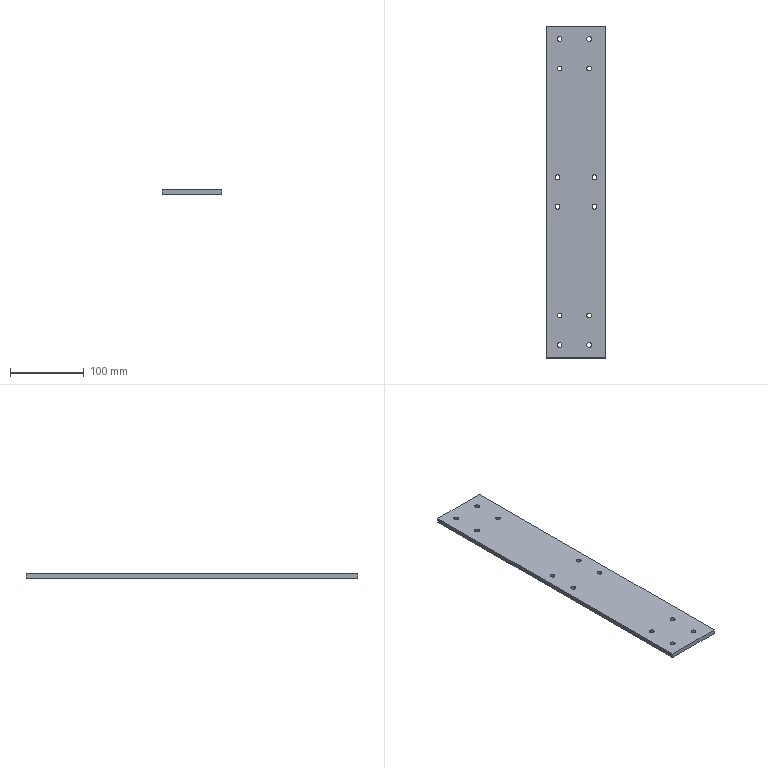Component | SolidWorks | DC-Motor-115-2 | 1 solid | 30 faces | box 80 x 450 x 6 mm | volume 213611 mm3 | cylinder 24 | plane 6 | commonest cylinder face diameters 6.5 x24
build123d program:
from build123d import *

# Parameters (mm, degrees)
SKETCH1_W                  = 450
SKETCH1_H                  = 80
BOSS_EXTRUDE1_DEPTH        = 3
F_6_5_6_5_DIAMETER_HOLE1_D = 6.5
F_6_5_6_5_DIAMETER_HOLE2_D = 6.5


with BuildPart() as part:
    # Sketch1 → Boss-Extrude1 (new, symmetric)
    with BuildSketch(Plane.XY):
        Rectangle(SKETCH1_W, SKETCH1_H)
    extrude(amount=BOSS_EXTRUDE1_DEPTH, both=True)

    # 6.5 _6.5_ Diameter Hole1 (through all)
    with Locations(Plane(origin=(0, 0, -3), x_dir=(-1, 0, 0), z_dir=(0, 0, -1))):
        with Locations((-167.5, -22.215), (-207.5, -22.215), (-207.5, 17.785), (-167.5, 17.785), (167.5, -22.215), (207.5, -22.215), (207.5, 17.785), (167.5, 17.785)):
            Hole(F_6_5_6_5_DIAMETER_HOLE1_D / 2)

    # 6.5 _6.5_ Diameter Hole2 (through all)
    with Locations(Plane(origin=(0, 0, -3), x_dir=(-1, 0, 0), z_dir=(0, 0, -1))):
        with Locations((20, -25), (-20, -25), (20, 25), (-20, 25)):
            Hole(F_6_5_6_5_DIAMETER_HOLE2_D / 2)


solid = part.part

# Placed as in the assembly
solid = solid.moved(Location((402.208, 14.301, -413), (0, 0, -90)))
STEP:
#1=CARTESIAN_POINT('',(14.851,1.222,-16.142));
#2=VERTEX_POINT('',#1);
#3=CARTESIAN_POINT('',(14.851,1.478,-16.142));
#4=VERTEX_POINT('',#3);
#5=CARTESIAN_POINT('',(14.851,1.35,-16.142));
#6=DIRECTION('',(0.,0.,-1.));
#7=DIRECTION('',(0.,1.,0.));
#8=AXIS2_PLACEMENT_3D('',#5,#6,#7);
#9=CIRCLE('',#8,0.128);
#10=EDGE_CURVE('',#2,#4,#9,.T.);
#11=ORIENTED_EDGE('',*,*,#10,.F.);
#12=CARTESIAN_POINT('',(14.851,1.222,-16.378));
#13=VERTEX_POINT('',#12);
#14=CARTESIAN_POINT('',(14.851,1.222,-16.378));
#15=DIRECTION('',(0.,0.,-1.));
#16=VECTOR('',#15,39.37);
#17=LINE('',#14,#16);
#18=EDGE_CURVE('',#2,#13,#17,.T.);
#19=ORIENTED_EDGE('',*,*,#18,.T.);
#20=CARTESIAN_POINT('',(14.851,1.478,-16.378));
#21=VERTEX_POINT('',#20);
#22=CARTESIAN_POINT('',(14.851,1.35,-16.378));
#23=DIRECTION('',(0.,0.,-1.));
#24=DIRECTION('',(0.,1.,0.));
#25=AXIS2_PLACEMENT_3D('',#22,#23,#24);
#26=CIRCLE('',#25,0.128);
#27=EDGE_CURVE('',#13,#21,#26,.T.);
#28=ORIENTED_EDGE('',*,*,#27,.T.);
#29=CARTESIAN_POINT('',(14.851,1.478,-16.378));
#30=DIRECTION('',(0.,0.,-1.));
#31=VECTOR('',#30,39.37);
#32=LINE('',#29,#31);
#33=EDGE_CURVE('',#4,#21,#32,.T.);
#34=ORIENTED_EDGE('',*,*,#33,.F.);
#35=EDGE_LOOP('',(#11,#19,#28,#34));
#36=FACE_OUTER_BOUND('',#35,.T.);
#37=CARTESIAN_POINT('',(14.851,1.35,-16.378));
#38=DIRECTION('',(0.,0.,-1.));
#39=DIRECTION('',(0.,1.,0.));
#40=AXIS2_PLACEMENT_3D('',#37,#38,#39);
#41=CYLINDRICAL_SURFACE('',#40,0.128);
#42=ADVANCED_FACE('',(#36),#41,.F.);
#43=CARTESIAN_POINT('',(14.851,-0.3523,-16.142));
#44=VERTEX_POINT('',#43);
#45=CARTESIAN_POINT('',(14.851,-0.09641,-16.142));
#46=VERTEX_POINT('',#45);
#47=CARTESIAN_POINT('',(14.851,-0.2244,-16.142));
#48=DIRECTION('',(0.,0.,-1.));
#49=DIRECTION('',(0.,1.,0.));
#50=AXIS2_PLACEMENT_3D('',#47,#48,#49);
#51=CIRCLE('',#50,0.128);
#52=EDGE_CURVE('',#44,#46,#51,.T.);
#53=ORIENTED_EDGE('',*,*,#52,.F.);
#54=CARTESIAN_POINT('',(14.851,-0.3523,-16.378));
#55=VERTEX_POINT('',#54);
#56=CARTESIAN_POINT('',(14.851,-0.3523,-16.378));
#57=DIRECTION('',(0.,0.,-1.));
#58=VECTOR('',#57,39.37);
#59=LINE('',#56,#58);
#60=EDGE_CURVE('',#44,#55,#59,.T.);
#61=ORIENTED_EDGE('',*,*,#60,.T.);
#62=CARTESIAN_POINT('',(14.851,-0.09641,-16.378));
#63=VERTEX_POINT('',#62);
#64=CARTESIAN_POINT('',(14.851,-0.2244,-16.378));
#65=DIRECTION('',(0.,0.,-1.));
#66=DIRECTION('',(0.,1.,0.));
#67=AXIS2_PLACEMENT_3D('',#64,#65,#66);
#68=CIRCLE('',#67,0.128);
#69=EDGE_CURVE('',#55,#63,#68,.T.);
#70=ORIENTED_EDGE('',*,*,#69,.T.);
#71=CARTESIAN_POINT('',(14.851,-0.09641,-16.378));
#72=DIRECTION('',(0.,0.,-1.));
#73=VECTOR('',#72,39.37);
#74=LINE('',#71,#73);
#75=EDGE_CURVE('',#46,#63,#74,.T.);
#76=ORIENTED_EDGE('',*,*,#75,.F.);
#77=EDGE_LOOP('',(#53,#61,#70,#76));
#78=FACE_OUTER_BOUND('',#77,.T.);
#79=CARTESIAN_POINT('',(14.851,-0.2244,-16.378));
#80=DIRECTION('',(0.,0.,-1.));
#81=DIRECTION('',(0.,1.,0.));
#82=AXIS2_PLACEMENT_3D('',#79,#80,#81);
#83=CYLINDRICAL_SURFACE('',#82,0.128);
#84=ADVANCED_FACE('',(#78),#83,.F.);
#85=CARTESIAN_POINT('',(16.819,1.222,-16.142));
#86=VERTEX_POINT('',#85);
#87=CARTESIAN_POINT('',(16.819,1.478,-16.142));
#88=VERTEX_POINT('',#87);
#89=CARTESIAN_POINT('',(16.819,1.35,-16.142));
#90=DIRECTION('',(0.,0.,-1.));
#91=DIRECTION('',(0.,1.,0.));
#92=AXIS2_PLACEMENT_3D('',#89,#90,#91);
#93=CIRCLE('',#92,0.128);
#94=EDGE_CURVE('',#86,#88,#93,.T.);
#95=ORIENTED_EDGE('',*,*,#94,.F.);
#96=CARTESIAN_POINT('',(16.819,1.222,-16.378));
#97=VERTEX_POINT('',#96);
#98=CARTESIAN_POINT('',(16.819,1.222,-16.378));
#99=DIRECTION('',(0.,0.,-1.));
#100=VECTOR('',#99,39.37);
#101=LINE('',#98,#100);
#102=EDGE_CURVE('',#86,#97,#101,.T.);
#103=ORIENTED_EDGE('',*,*,#102,.T.);
#104=CARTESIAN_POINT('',(16.819,1.478,-16.378));
#105=VERTEX_POINT('',#104);
#106=CARTESIAN_POINT('',(16.819,1.35,-16.378));
#107=DIRECTION('',(0.,0.,-1.));
#108=DIRECTION('',(0.,1.,0.));
#109=AXIS2_PLACEMENT_3D('',#106,#107,#108);
#110=CIRCLE('',#109,0.128);
#111=EDGE_CURVE('',#97,#105,#110,.T.);
#112=ORIENTED_EDGE('',*,*,#111,.T.);
#113=CARTESIAN_POINT('',(16.819,1.478,-16.378));
#114=DIRECTION('',(0.,0.,-1.));
#115=VECTOR('',#114,39.37);
#116=LINE('',#113,#115);
#117=EDGE_CURVE('',#88,#105,#116,.T.);
#118=ORIENTED_EDGE('',*,*,#117,.F.);
#119=EDGE_LOOP('',(#95,#103,#112,#118));
#120=FACE_OUTER_BOUND('',#119,.T.);
#121=CARTESIAN_POINT('',(16.819,1.35,-16.378));
#122=DIRECTION('',(0.,0.,-1.));
#123=DIRECTION('',(0.,1.,0.));
#124=AXIS2_PLACEMENT_3D('',#121,#122,#123);
#125=CYLINDRICAL_SURFACE('',#124,0.128);
#126=ADVANCED_FACE('',(#120),#125,.F.);
#127=CARTESIAN_POINT('',(16.819,-0.3523,-16.142));
#128=VERTEX_POINT('',#127);
#129=CARTESIAN_POINT('',(16.819,-0.09641,-16.142));
#130=VERTEX_POINT('',#129);
#131=CARTESIAN_POINT('',(16.819,-0.2244,-16.142));
#132=DIRECTION('',(0.,0.,-1.));
#133=DIRECTION('',(0.,1.,0.));
#134=AXIS2_PLACEMENT_3D('',#131,#132,#133);
#135=CIRCLE('',#134,0.128);
#136=EDGE_CURVE('',#128,#130,#135,.T.);
#137=ORIENTED_EDGE('',*,*,#136,.F.);
#138=CARTESIAN_POINT('',(16.819,-0.3523,-16.378));
#139=VERTEX_POINT('',#138);
#140=CARTESIAN_POINT('',(16.819,-0.3523,-16.378));
#141=DIRECTION('',(0.,0.,-1.));
#142=VECTOR('',#141,39.37);
#143=LINE('',#140,#142);
#144=EDGE_CURVE('',#128,#139,#143,.T.);
#145=ORIENTED_EDGE('',*,*,#144,.T.);
#146=CARTESIAN_POINT('',(16.819,-0.09641,-16.378));
#147=VERTEX_POINT('',#146);
#148=CARTESIAN_POINT('',(16.819,-0.2244,-16.378));
#149=DIRECTION('',(0.,0.,-1.));
#150=DIRECTION('',(0.,1.,0.));
#151=AXIS2_PLACEMENT_3D('',#148,#149,#150);
#152=CIRCLE('',#151,0.128);
#153=EDGE_CURVE('',#139,#147,#152,.T.);
#154=ORIENTED_EDGE('',*,*,#153,.T.);
#155=CARTESIAN_POINT('',(16.819,-0.09641,-16.378));
#156=DIRECTION('',(0.,0.,-1.));
#157=VECTOR('',#156,39.37);
#158=LINE('',#155,#157);
#159=EDGE_CURVE('',#130,#147,#158,.T.);
#160=ORIENTED_EDGE('',*,*,#159,.F.);
#161=EDGE_LOOP('',(#137,#145,#154,#160));
#162=FACE_OUTER_BOUND('',#161,.T.);
#163=CARTESIAN_POINT('',(16.819,-0.2244,-16.378));
#164=DIRECTION('',(0.,0.,-1.));
#165=DIRECTION('',(0.,1.,0.));
#166=AXIS2_PLACEMENT_3D('',#163,#164,#165);
#167=CYLINDRICAL_SURFACE('',#166,0.128);
#168=ADVANCED_FACE('',(#162),#167,.F.);
#169=CARTESIAN_POINT('',(14.96,-6.159,-16.142));
#170=VERTEX_POINT('',#169);
#171=CARTESIAN_POINT('',(14.96,-5.903,-16.142));
#172=VERTEX_POINT('',#171);
#173=CARTESIAN_POINT('',(14.96,-6.031,-16.142));
#174=DIRECTION('',(0.,0.,-1.));
#175=DIRECTION('',(0.,1.,0.));
#176=AXIS2_PLACEMENT_3D('',#173,#174,#175);
#177=CIRCLE('',#176,0.128);
#178=EDGE_CURVE('',#170,#172,#177,.T.);
#179=ORIENTED_EDGE('',*,*,#178,.F.);
#180=CARTESIAN_POINT('',(14.96,-6.159,-16.378));
#181=VERTEX_POINT('',#180);
#182=CARTESIAN_POINT('',(14.96,-6.159,-16.378));
#183=DIRECTION('',(0.,0.,-1.));
#184=VECTOR('',#183,39.37);
#185=LINE('',#182,#184);
#186=EDGE_CURVE('',#170,#181,#185,.T.);
#187=ORIENTED_EDGE('',*,*,#186,.T.);
#188=CARTESIAN_POINT('',(14.96,-5.903,-16.378));
#189=VERTEX_POINT('',#188);
#190=CARTESIAN_POINT('',(14.96,-6.031,-16.378));
#191=DIRECTION('',(0.,0.,-1.));
#192=DIRECTION('',(0.,1.,0.));
#193=AXIS2_PLACEMENT_3D('',#190,#191,#192);
#194=CIRCLE('',#193,0.128);
#195=EDGE_CURVE('',#181,#189,#194,.T.);
#196=ORIENTED_EDGE('',*,*,#195,.T.);
#197=CARTESIAN_POINT('',(14.96,-5.903,-16.378));
#198=DIRECTION('',(0.,0.,-1.));
#199=VECTOR('',#198,39.37);
#200=LINE('',#197,#199);
#201=EDGE_CURVE('',#172,#189,#200,.T.);
#202=ORIENTED_EDGE('',*,*,#201,.F.);
#203=EDGE_LOOP('',(#179,#187,#196,#202));
#204=FACE_OUTER_BOUND('',#203,.T.);
#205=CARTESIAN_POINT('',(14.96,-6.031,-16.378));
#206=DIRECTION('',(0.,0.,-1.));
#207=DIRECTION('',(0.,1.,0.));
#208=AXIS2_PLACEMENT_3D('',#205,#206,#207);
#209=CYLINDRICAL_SURFACE('',#208,0.128);
#210=ADVANCED_FACE('',(#204),#209,.F.);
#211=CARTESIAN_POINT('',(14.96,-7.734,-16.142));
#212=VERTEX_POINT('',#211);
#213=CARTESIAN_POINT('',(14.96,-7.478,-16.142));
#214=VERTEX_POINT('',#213);
#215=CARTESIAN_POINT('',(14.96,-7.606,-16.142));
#216=DIRECTION('',(0.,0.,-1.));
#217=DIRECTION('',(0.,1.,0.));
#218=AXIS2_PLACEMENT_3D('',#215,#216,#217);
#219=CIRCLE('',#218,0.128);
#220=EDGE_CURVE('',#212,#214,#219,.T.);
#221=ORIENTED_EDGE('',*,*,#220,.F.);
#222=CARTESIAN_POINT('',(14.96,-7.734,-16.378));
#223=VERTEX_POINT('',#222);
#224=CARTESIAN_POINT('',(14.96,-7.734,-16.378));
#225=DIRECTION('',(0.,0.,-1.));
#226=VECTOR('',#225,39.37);
#227=LINE('',#224,#226);
#228=EDGE_CURVE('',#212,#223,#227,.T.);
#229=ORIENTED_EDGE('',*,*,#228,.T.);
#230=CARTESIAN_POINT('',(14.96,-7.478,-16.378));
#231=VERTEX_POINT('',#230);
#232=CARTESIAN_POINT('',(14.96,-7.606,-16.378));
#233=DIRECTION('',(0.,0.,-1.));
#234=DIRECTION('',(0.,1.,0.));
#235=AXIS2_PLACEMENT_3D('',#232,#233,#234);
#236=CIRCLE('',#235,0.128);
#237=EDGE_CURVE('',#223,#231,#236,.T.);
#238=ORIENTED_EDGE('',*,*,#237,.T.);
#239=CARTESIAN_POINT('',(14.96,-7.478,-16.378));
#240=DIRECTION('',(0.,0.,-1.));
#241=VECTOR('',#240,39.37);
#242=LINE('',#239,#241);
#243=EDGE_CURVE('',#214,#231,#242,.T.);
#244=ORIENTED_EDGE('',*,*,#243,.F.);
#245=EDGE_LOOP('',(#221,#229,#238,#244));
#246=FACE_OUTER_BOUND('',#245,.T.);
#247=CARTESIAN_POINT('',(14.96,-7.606,-16.378));
#248=DIRECTION('',(0.,0.,-1.));
#249=DIRECTION('',(0.,1.,0.));
#250=AXIS2_PLACEMENT_3D('',#247,#248,#249);
#251=CYLINDRICAL_SURFACE('',#250,0.128);
#252=ADVANCED_FACE('',(#246),#251,.F.);
#253=CARTESIAN_POINT('',(16.535,-7.734,-16.142));
#254=VERTEX_POINT('',#253);
#255=CARTESIAN_POINT('',(16.535,-7.478,-16.142));
#256=VERTEX_POINT('',#255);
#257=CARTESIAN_POINT('',(16.535,-7.606,-16.142));
#258=DIRECTION('',(0.,0.,-1.));
#259=DIRECTION('',(0.,1.,0.));
#260=AXIS2_PLACEMENT_3D('',#257,#258,#259);
#261=CIRCLE('',#260,0.128);
#262=EDGE_CURVE('',#254,#256,#261,.T.);
#263=ORIENTED_EDGE('',*,*,#262,.F.);
#264=CARTESIAN_POINT('',(16.535,-7.734,-16.378));
#265=VERTEX_POINT('',#264);
#266=CARTESIAN_POINT('',(16.535,-7.734,-16.378));
#267=DIRECTION('',(0.,0.,-1.));
#268=VECTOR('',#267,39.37);
#269=LINE('',#266,#268);
#270=EDGE_CURVE('',#254,#265,#269,.T.);
#271=ORIENTED_EDGE('',*,*,#270,.T.);
#272=CARTESIAN_POINT('',(16.535,-7.478,-16.378));
#273=VERTEX_POINT('',#272);
#274=CARTESIAN_POINT('',(16.535,-7.606,-16.378));
#275=DIRECTION('',(0.,0.,-1.));
#276=DIRECTION('',(0.,1.,0.));
#277=AXIS2_PLACEMENT_3D('',#274,#275,#276);
#278=CIRCLE('',#277,0.128);
#279=EDGE_CURVE('',#265,#273,#278,.T.);
#280=ORIENTED_EDGE('',*,*,#279,.T.);
#281=CARTESIAN_POINT('',(16.535,-7.478,-16.378));
#282=DIRECTION('',(0.,0.,-1.));
#283=VECTOR('',#282,39.37);
#284=LINE('',#281,#283);
#285=EDGE_CURVE('',#256,#273,#284,.T.);
#286=ORIENTED_EDGE('',*,*,#285,.F.);
#287=EDGE_LOOP('',(#263,#271,#280,#286));
#288=FACE_OUTER_BOUND('',#287,.T.);
#289=CARTESIAN_POINT('',(16.535,-7.606,-16.378));
#290=DIRECTION('',(0.,0.,-1.));
#291=DIRECTION('',(0.,1.,0.));
#292=AXIS2_PLACEMENT_3D('',#289,#290,#291);
#293=CYLINDRICAL_SURFACE('',#292,0.128);
#294=ADVANCED_FACE('',(#288),#293,.F.);
#295=CARTESIAN_POINT('',(16.535,-6.159,-16.142));
#296=VERTEX_POINT('',#295);
#297=CARTESIAN_POINT('',(16.535,-5.903,-16.142));
#298=VERTEX_POINT('',#297);
#299=CARTESIAN_POINT('',(16.535,-6.031,-16.142));
#300=DIRECTION('',(0.,0.,-1.));
#301=DIRECTION('',(0.,1.,0.));
#302=AXIS2_PLACEMENT_3D('',#299,#300,#301);
#303=CIRCLE('',#302,0.128);
#304=EDGE_CURVE('',#296,#298,#303,.T.);
#305=ORIENTED_EDGE('',*,*,#304,.F.);
#306=CARTESIAN_POINT('',(16.535,-6.159,-16.378));
#307=VERTEX_POINT('',#306);
#308=CARTESIAN_POINT('',(16.535,-6.159,-16.378));
#309=DIRECTION('',(0.,0.,-1.));
#310=VECTOR('',#309,39.37);
#311=LINE('',#308,#310);
#312=EDGE_CURVE('',#296,#307,#311,.T.);
#313=ORIENTED_EDGE('',*,*,#312,.T.);
#314=CARTESIAN_POINT('',(16.535,-5.903,-16.378));
#315=VERTEX_POINT('',#314);
#316=CARTESIAN_POINT('',(16.535,-6.031,-16.378));
#317=DIRECTION('',(0.,0.,-1.));
#318=DIRECTION('',(0.,1.,0.));
#319=AXIS2_PLACEMENT_3D('',#316,#317,#318);
#320=CIRCLE('',#319,0.128);
#321=EDGE_CURVE('',#307,#315,#320,.T.);
#322=ORIENTED_EDGE('',*,*,#321,.T.);
#323=CARTESIAN_POINT('',(16.535,-5.903,-16.378));
#324=DIRECTION('',(0.,0.,-1.));
#325=VECTOR('',#324,39.37);
#326=LINE('',#323,#325);
#327=EDGE_CURVE('',#298,#315,#326,.T.);
#328=ORIENTED_EDGE('',*,*,#327,.F.);
#329=EDGE_LOOP('',(#305,#313,#322,#328));
#330=FACE_OUTER_BOUND('',#329,.T.);
#331=CARTESIAN_POINT('',(16.535,-6.031,-16.378));
#332=DIRECTION('',(0.,0.,-1.));
#333=DIRECTION('',(0.,1.,0.));
#334=AXIS2_PLACEMENT_3D('',#331,#332,#333);
#335=CYLINDRICAL_SURFACE('',#334,0.128);
#336=ADVANCED_FACE('',(#330),#335,.F.);
#337=CARTESIAN_POINT('',(14.96,7.03,-16.142));
#338=VERTEX_POINT('',#337);
#339=CARTESIAN_POINT('',(14.96,7.285,-16.142));
#340=VERTEX_POINT('',#339);
#341=CARTESIAN_POINT('',(14.96,7.158,-16.142));
#342=DIRECTION('',(0.,0.,-1.));
#343=DIRECTION('',(0.,1.,0.));
#344=AXIS2_PLACEMENT_3D('',#341,#342,#343);
#345=CIRCLE('',#344,0.128);
#346=EDGE_CURVE('',#338,#340,#345,.T.);
#347=ORIENTED_EDGE('',*,*,#346,.F.);
#348=CARTESIAN_POINT('',(14.96,7.03,-16.378));
#349=VERTEX_POINT('',#348);
#350=CARTESIAN_POINT('',(14.96,7.03,-16.378));
#351=DIRECTION('',(0.,0.,-1.));
#352=VECTOR('',#351,39.37);
#353=LINE('',#350,#352);
#354=EDGE_CURVE('',#338,#349,#353,.T.);
#355=ORIENTED_EDGE('',*,*,#354,.T.);
#356=CARTESIAN_POINT('',(14.96,7.285,-16.378));
#357=VERTEX_POINT('',#356);
#358=CARTESIAN_POINT('',(14.96,7.158,-16.378));
#359=DIRECTION('',(0.,0.,-1.));
#360=DIRECTION('',(0.,1.,0.));
#361=AXIS2_PLACEMENT_3D('',#358,#359,#360);
#362=CIRCLE('',#361,0.128);
#363=EDGE_CURVE('',#349,#357,#362,.T.);
#364=ORIENTED_EDGE('',*,*,#363,.T.);
#365=CARTESIAN_POINT('',(14.96,7.285,-16.378));
#366=DIRECTION('',(0.,0.,-1.));
#367=VECTOR('',#366,39.37);
#368=LINE('',#365,#367);
#369=EDGE_CURVE('',#340,#357,#368,.T.);
#370=ORIENTED_EDGE('',*,*,#369,.F.);
#371=EDGE_LOOP('',(#347,#355,#364,#370));
#372=FACE_OUTER_BOUND('',#371,.T.);
#373=CARTESIAN_POINT('',(14.96,7.158,-16.378));
#374=DIRECTION('',(0.,0.,-1.));
#375=DIRECTION('',(0.,1.,0.));
#376=AXIS2_PLACEMENT_3D('',#373,#374,#375);
#377=CYLINDRICAL_SURFACE('',#376,0.128);
#378=ADVANCED_FACE('',(#372),#377,.F.);
#379=CARTESIAN_POINT('',(14.96,8.604,-16.142));
#380=VERTEX_POINT('',#379);
#381=CARTESIAN_POINT('',(14.96,8.86,-16.142));
#382=VERTEX_POINT('',#381);
#383=CARTESIAN_POINT('',(14.96,8.732,-16.142));
#384=DIRECTION('',(0.,0.,-1.));
#385=DIRECTION('',(0.,1.,0.));
#386=AXIS2_PLACEMENT_3D('',#383,#384,#385);
#387=CIRCLE('',#386,0.128);
#388=EDGE_CURVE('',#380,#382,#387,.T.);
#389=ORIENTED_EDGE('',*,*,#388,.F.);
#390=CARTESIAN_POINT('',(14.96,8.604,-16.378));
#391=VERTEX_POINT('',#390);
#392=CARTESIAN_POINT('',(14.96,8.604,-16.378));
#393=DIRECTION('',(0.,0.,-1.));
#394=VECTOR('',#393,39.37);
#395=LINE('',#392,#394);
#396=EDGE_CURVE('',#380,#391,#395,.T.);
#397=ORIENTED_EDGE('',*,*,#396,.T.);
#398=CARTESIAN_POINT('',(14.96,8.86,-16.378));
#399=VERTEX_POINT('',#398);
#400=CARTESIAN_POINT('',(14.96,8.732,-16.378));
#401=DIRECTION('',(0.,0.,-1.));
#402=DIRECTION('',(0.,1.,0.));
#403=AXIS2_PLACEMENT_3D('',#400,#401,#402);
#404=CIRCLE('',#403,0.128);
#405=EDGE_CURVE('',#391,#399,#404,.T.);
#406=ORIENTED_EDGE('',*,*,#405,.T.);
#407=CARTESIAN_POINT('',(14.96,8.86,-16.378));
#408=DIRECTION('',(0.,0.,-1.));
#409=VECTOR('',#408,39.37);
#410=LINE('',#407,#409);
#411=EDGE_CURVE('',#382,#399,#410,.T.);
#412=ORIENTED_EDGE('',*,*,#411,.F.);
#413=EDGE_LOOP('',(#389,#397,#406,#412));
#414=FACE_OUTER_BOUND('',#413,.T.);
#415=CARTESIAN_POINT('',(14.96,8.732,-16.378));
#416=DIRECTION('',(0.,0.,-1.));
#417=DIRECTION('',(0.,1.,0.));
#418=AXIS2_PLACEMENT_3D('',#415,#416,#417);
#419=CYLINDRICAL_SURFACE('',#418,0.128);
#420=ADVANCED_FACE('',(#414),#419,.F.);
#421=CARTESIAN_POINT('',(16.535,8.604,-16.142));
#422=VERTEX_POINT('',#421);
#423=CARTESIAN_POINT('',(16.535,8.86,-16.142));
#424=VERTEX_POINT('',#423);
#425=CARTESIAN_POINT('',(16.535,8.732,-16.142));
#426=DIRECTION('',(0.,0.,-1.));
#427=DIRECTION('',(0.,1.,0.));
#428=AXIS2_PLACEMENT_3D('',#425,#426,#427);
#429=CIRCLE('',#428,0.128);
#430=EDGE_CURVE('',#422,#424,#429,.T.);
#431=ORIENTED_EDGE('',*,*,#430,.F.);
#432=CARTESIAN_POINT('',(16.535,8.604,-16.378));
#433=VERTEX_POINT('',#432);
#434=CARTESIAN_POINT('',(16.535,8.604,-16.378));
#435=DIRECTION('',(0.,0.,-1.));
#436=VECTOR('',#435,39.37);
#437=LINE('',#434,#436);
#438=EDGE_CURVE('',#422,#433,#437,.T.);
#439=ORIENTED_EDGE('',*,*,#438,.T.);
#440=CARTESIAN_POINT('',(16.535,8.86,-16.378));
#441=VERTEX_POINT('',#440);
#442=CARTESIAN_POINT('',(16.535,8.732,-16.378));
#443=DIRECTION('',(0.,0.,-1.));
#444=DIRECTION('',(0.,1.,0.));
#445=AXIS2_PLACEMENT_3D('',#442,#443,#444);
#446=CIRCLE('',#445,0.128);
#447=EDGE_CURVE('',#433,#441,#446,.T.);
#448=ORIENTED_EDGE('',*,*,#447,.T.);
#449=CARTESIAN_POINT('',(16.535,8.86,-16.378));
#450=DIRECTION('',(0.,0.,-1.));
#451=VECTOR('',#450,39.37);
#452=LINE('',#449,#451);
#453=EDGE_CURVE('',#424,#441,#452,.T.);
#454=ORIENTED_EDGE('',*,*,#453,.F.);
#455=EDGE_LOOP('',(#431,#439,#448,#454));
#456=FACE_OUTER_BOUND('',#455,.T.);
#457=CARTESIAN_POINT('',(16.535,8.732,-16.378));
#458=DIRECTION('',(0.,0.,-1.));
#459=DIRECTION('',(0.,1.,0.));
#460=AXIS2_PLACEMENT_3D('',#457,#458,#459);
#461=CYLINDRICAL_SURFACE('',#460,0.128);
#462=ADVANCED_FACE('',(#456),#461,.F.);
#463=CARTESIAN_POINT('',(16.535,7.03,-16.142));
#464=VERTEX_POINT('',#463);
#465=CARTESIAN_POINT('',(16.535,7.285,-16.142));
#466=VERTEX_POINT('',#465);
#467=CARTESIAN_POINT('',(16.535,7.158,-16.142));
#468=DIRECTION('',(0.,0.,-1.));
#469=DIRECTION('',(0.,1.,0.));
#470=AXIS2_PLACEMENT_3D('',#467,#468,#469);
#471=CIRCLE('',#470,0.128);
#472=EDGE_CURVE('',#464,#466,#471,.T.);
#473=ORIENTED_EDGE('',*,*,#472,.F.);
#474=CARTESIAN_POINT('',(16.535,7.03,-16.378));
#475=VERTEX_POINT('',#474);
#476=CARTESIAN_POINT('',(16.535,7.03,-16.378));
#477=DIRECTION('',(0.,0.,-1.));
#478=VECTOR('',#477,39.37);
#479=LINE('',#476,#478);
#480=EDGE_CURVE('',#464,#475,#479,.T.);
#481=ORIENTED_EDGE('',*,*,#480,.T.);
#482=CARTESIAN_POINT('',(16.535,7.285,-16.378));
#483=VERTEX_POINT('',#482);
#484=CARTESIAN_POINT('',(16.535,7.158,-16.378));
#485=DIRECTION('',(0.,0.,-1.));
#486=DIRECTION('',(0.,1.,0.));
#487=AXIS2_PLACEMENT_3D('',#484,#485,#486);
#488=CIRCLE('',#487,0.128);
#489=EDGE_CURVE('',#475,#483,#488,.T.);
#490=ORIENTED_EDGE('',*,*,#489,.T.);
#491=CARTESIAN_POINT('',(16.535,7.285,-16.378));
#492=DIRECTION('',(0.,0.,-1.));
#493=VECTOR('',#492,39.37);
#494=LINE('',#491,#493);
#495=EDGE_CURVE('',#466,#483,#494,.T.);
#496=ORIENTED_EDGE('',*,*,#495,.F.);
#497=EDGE_LOOP('',(#473,#481,#490,#496));
#498=FACE_OUTER_BOUND('',#497,.T.);
#499=CARTESIAN_POINT('',(16.535,7.158,-16.378));
#500=DIRECTION('',(0.,0.,-1.));
#501=DIRECTION('',(0.,1.,0.));
#502=AXIS2_PLACEMENT_3D('',#499,#500,#501);
#503=CYLINDRICAL_SURFACE('',#502,0.128);
#504=ADVANCED_FACE('',(#498),#503,.F.);
#505=CARTESIAN_POINT('',(14.851,1.35,-16.378));
#506=DIRECTION('',(0.,0.,-1.));
#507=DIRECTION('',(0.,1.,0.));
#508=AXIS2_PLACEMENT_3D('',#505,#506,#507);
#509=CIRCLE('',#508,0.128);
#510=EDGE_CURVE('',#21,#13,#509,.T.);
#511=ORIENTED_EDGE('',*,*,#510,.F.);
#512=ORIENTED_EDGE('',*,*,#27,.F.);
#513=EDGE_LOOP('',(#511,#512));
#514=FACE_BOUND('',#513,.T.);
#515=CARTESIAN_POINT('',(14.851,-0.2244,-16.378));
#516=DIRECTION('',(0.,0.,-1.));
#517=DIRECTION('',(0.,1.,0.));
#518=AXIS2_PLACEMENT_3D('',#515,#516,#517);
#519=CIRCLE('',#518,0.128);
#520=EDGE_CURVE('',#63,#55,#519,.T.);
#521=ORIENTED_EDGE('',*,*,#520,.F.);
#522=ORIENTED_EDGE('',*,*,#69,.F.);
#523=EDGE_LOOP('',(#521,#522));
#524=FACE_BOUND('',#523,.T.);
#525=CARTESIAN_POINT('',(16.819,1.35,-16.378));
#526=DIRECTION('',(0.,0.,-1.));
#527=DIRECTION('',(0.,1.,0.));
#528=AXIS2_PLACEMENT_3D('',#525,#526,#527);
#529=CIRCLE('',#528,0.128);
#530=EDGE_CURVE('',#105,#97,#529,.T.);
#531=ORIENTED_EDGE('',*,*,#530,.F.);
#532=ORIENTED_EDGE('',*,*,#111,.F.);
#533=EDGE_LOOP('',(#531,#532));
#534=FACE_BOUND('',#533,.T.);
#535=CARTESIAN_POINT('',(16.819,-0.2244,-16.378));
#536=DIRECTION('',(0.,0.,-1.));
#537=DIRECTION('',(0.,1.,0.));
#538=AXIS2_PLACEMENT_3D('',#535,#536,#537);
#539=CIRCLE('',#538,0.128);
#540=EDGE_CURVE('',#147,#139,#539,.T.);
#541=ORIENTED_EDGE('',*,*,#540,.F.);
#542=ORIENTED_EDGE('',*,*,#153,.F.);
#543=EDGE_LOOP('',(#541,#542));
#544=FACE_BOUND('',#543,.T.);
#545=CARTESIAN_POINT('',(14.96,-6.031,-16.378));
#546=DIRECTION('',(0.,0.,-1.));
#547=DIRECTION('',(0.,1.,0.));
#548=AXIS2_PLACEMENT_3D('',#545,#546,#547);
#549=CIRCLE('',#548,0.128);
#550=EDGE_CURVE('',#189,#181,#549,.T.);
#551=ORIENTED_EDGE('',*,*,#550,.F.);
#552=ORIENTED_EDGE('',*,*,#195,.F.);
#553=EDGE_LOOP('',(#551,#552));
#554=FACE_BOUND('',#553,.T.);
#555=CARTESIAN_POINT('',(16.535,-7.606,-16.378));
#556=DIRECTION('',(0.,0.,-1.));
#557=DIRECTION('',(0.,1.,0.));
#558=AXIS2_PLACEMENT_3D('',#555,#556,#557);
#559=CIRCLE('',#558,0.128);
#560=EDGE_CURVE('',#273,#265,#559,.T.);
#561=ORIENTED_EDGE('',*,*,#560,.F.);
#562=ORIENTED_EDGE('',*,*,#279,.F.);
#563=EDGE_LOOP('',(#561,#562));
#564=FACE_BOUND('',#563,.T.);
#565=CARTESIAN_POINT('',(16.535,-6.031,-16.378));
#566=DIRECTION('',(0.,0.,-1.));
#567=DIRECTION('',(0.,1.,0.));
#568=AXIS2_PLACEMENT_3D('',#565,#566,#567);
#569=CIRCLE('',#568,0.128);
#570=EDGE_CURVE('',#315,#307,#569,.T.);
#571=ORIENTED_EDGE('',*,*,#570,.F.);
#572=ORIENTED_EDGE('',*,*,#321,.F.);
#573=EDGE_LOOP('',(#571,#572));
#574=FACE_BOUND('',#573,.T.);
#575=CARTESIAN_POINT('',(14.96,8.732,-16.378));
#576=DIRECTION('',(0.,0.,-1.));
#577=DIRECTION('',(0.,1.,0.));
#578=AXIS2_PLACEMENT_3D('',#575,#576,#577);
#579=CIRCLE('',#578,0.128);
#580=EDGE_CURVE('',#399,#391,#579,.T.);
#581=ORIENTED_EDGE('',*,*,#580,.F.);
#582=ORIENTED_EDGE('',*,*,#405,.F.);
#583=EDGE_LOOP('',(#581,#582));
#584=FACE_BOUND('',#583,.T.);
#585=CARTESIAN_POINT('',(16.535,8.732,-16.378));
#586=DIRECTION('',(0.,0.,-1.));
#587=DIRECTION('',(0.,1.,0.));
#588=AXIS2_PLACEMENT_3D('',#585,#586,#587);
#589=CIRCLE('',#588,0.128);
#590=EDGE_CURVE('',#441,#433,#589,.T.);
#591=ORIENTED_EDGE('',*,*,#590,.F.);
#592=ORIENTED_EDGE('',*,*,#447,.F.);
#593=EDGE_LOOP('',(#591,#592));
#594=FACE_BOUND('',#593,.T.);
#595=CARTESIAN_POINT('',(16.535,7.158,-16.378));
#596=DIRECTION('',(0.,0.,-1.));
#597=DIRECTION('',(0.,1.,0.));
#598=AXIS2_PLACEMENT_3D('',#595,#596,#597);
#599=CIRCLE('',#598,0.128);
#600=EDGE_CURVE('',#483,#475,#599,.T.);
#601=ORIENTED_EDGE('',*,*,#600,.F.);
#602=ORIENTED_EDGE('',*,*,#489,.F.);
#603=EDGE_LOOP('',(#601,#602));
#604=FACE_BOUND('',#603,.T.);
#605=CARTESIAN_POINT('',(17.41,9.421,-16.378));
#606=VERTEX_POINT('',#605);
#607=CARTESIAN_POINT('',(14.26,9.421,-16.378));
#608=VERTEX_POINT('',#607);
#609=CARTESIAN_POINT('',(14.26,9.421,-16.378));
#610=DIRECTION('',(-1.,0.,-0.));
#611=VECTOR('',#610,39.37);
#612=LINE('',#609,#611);
#613=EDGE_CURVE('',#606,#608,#612,.T.);
#614=ORIENTED_EDGE('',*,*,#613,.F.);
#615=CARTESIAN_POINT('',(17.41,-8.295,-16.378));
#616=VERTEX_POINT('',#615);
#617=CARTESIAN_POINT('',(17.41,-8.295,-16.378));
#618=DIRECTION('',(-0.,1.,0.));
#619=VECTOR('',#618,39.37);
#620=LINE('',#617,#619);
#621=EDGE_CURVE('',#616,#606,#620,.T.);
#622=ORIENTED_EDGE('',*,*,#621,.F.);
#623=CARTESIAN_POINT('',(14.26,-8.295,-16.378));
#624=VERTEX_POINT('',#623);
#625=CARTESIAN_POINT('',(14.26,-8.295,-16.378));
#626=DIRECTION('',(1.,-0.,0.));
#627=VECTOR('',#626,39.37);
#628=LINE('',#625,#627);
#629=EDGE_CURVE('',#624,#616,#628,.T.);
#630=ORIENTED_EDGE('',*,*,#629,.F.);
#631=CARTESIAN_POINT('',(14.26,-8.295,-16.378));
#632=DIRECTION('',(0.,-1.,-0.));
#633=VECTOR('',#632,39.37);
#634=LINE('',#631,#633);
#635=EDGE_CURVE('',#608,#624,#634,.T.);
#636=ORIENTED_EDGE('',*,*,#635,.F.);
#637=EDGE_LOOP('',(#614,#622,#630,#636));
#638=FACE_OUTER_BOUND('',#637,.T.);
#639=CARTESIAN_POINT('',(14.96,7.158,-16.378));
#640=DIRECTION('',(0.,0.,-1.));
#641=DIRECTION('',(0.,1.,0.));
#642=AXIS2_PLACEMENT_3D('',#639,#640,#641);
#643=CIRCLE('',#642,0.128);
#644=EDGE_CURVE('',#357,#349,#643,.T.);
#645=ORIENTED_EDGE('',*,*,#644,.F.);
#646=ORIENTED_EDGE('',*,*,#363,.F.);
#647=EDGE_LOOP('',(#645,#646));
#648=FACE_BOUND('',#647,.T.);
#649=CARTESIAN_POINT('',(14.96,-7.606,-16.378));
#650=DIRECTION('',(0.,0.,-1.));
#651=DIRECTION('',(0.,1.,0.));
#652=AXIS2_PLACEMENT_3D('',#649,#650,#651);
#653=CIRCLE('',#652,0.128);
#654=EDGE_CURVE('',#231,#223,#653,.T.);
#655=ORIENTED_EDGE('',*,*,#654,.F.);
#656=ORIENTED_EDGE('',*,*,#237,.F.);
#657=EDGE_LOOP('',(#655,#656));
#658=FACE_BOUND('',#657,.T.);
#659=CARTESIAN_POINT('',(15.835,0.563,-16.378));
#660=DIRECTION('',(-0.,-0.,1.));
#661=DIRECTION('',(-0.,-1.,-0.));
#662=AXIS2_PLACEMENT_3D('',#659,#660,#661);
#663=PLANE('',#662);
#664=ADVANCED_FACE('',(#514,#524,#534,#544,#554,#564,#574,#584,#594,#604,#638,#648,#658),#663,.F.);
#665=CARTESIAN_POINT('',(14.851,1.35,-16.142));
#666=DIRECTION('',(0.,0.,-1.));
#667=DIRECTION('',(0.,1.,0.));
#668=AXIS2_PLACEMENT_3D('',#665,#666,#667);
#669=CIRCLE('',#668,0.128);
#670=EDGE_CURVE('',#4,#2,#669,.T.);
#671=ORIENTED_EDGE('',*,*,#670,.T.);
#672=ORIENTED_EDGE('',*,*,#10,.T.);
#673=EDGE_LOOP('',(#671,#672));
#674=FACE_BOUND('',#673,.T.);
#675=CARTESIAN_POINT('',(14.851,-0.2244,-16.142));
#676=DIRECTION('',(0.,0.,-1.));
#677=DIRECTION('',(0.,1.,0.));
#678=AXIS2_PLACEMENT_3D('',#675,#676,#677);
#679=CIRCLE('',#678,0.128);
#680=EDGE_CURVE('',#46,#44,#679,.T.);
#681=ORIENTED_EDGE('',*,*,#680,.T.);
#682=ORIENTED_EDGE('',*,*,#52,.T.);
#683=EDGE_LOOP('',(#681,#682));
#684=FACE_BOUND('',#683,.T.);
#685=CARTESIAN_POINT('',(16.819,1.35,-16.142));
#686=DIRECTION('',(0.,0.,-1.));
#687=DIRECTION('',(0.,1.,0.));
#688=AXIS2_PLACEMENT_3D('',#685,#686,#687);
#689=CIRCLE('',#688,0.128);
#690=EDGE_CURVE('',#88,#86,#689,.T.);
#691=ORIENTED_EDGE('',*,*,#690,.T.);
#692=ORIENTED_EDGE('',*,*,#94,.T.);
#693=EDGE_LOOP('',(#691,#692));
#694=FACE_BOUND('',#693,.T.);
#695=CARTESIAN_POINT('',(16.819,-0.2244,-16.142));
#696=DIRECTION('',(0.,0.,-1.));
#697=DIRECTION('',(0.,1.,0.));
#698=AXIS2_PLACEMENT_3D('',#695,#696,#697);
#699=CIRCLE('',#698,0.128);
#700=EDGE_CURVE('',#130,#128,#699,.T.);
#701=ORIENTED_EDGE('',*,*,#700,.T.);
#702=ORIENTED_EDGE('',*,*,#136,.T.);
#703=EDGE_LOOP('',(#701,#702));
#704=FACE_BOUND('',#703,.T.);
#705=CARTESIAN_POINT('',(14.96,-6.031,-16.142));
#706=DIRECTION('',(0.,0.,-1.));
#707=DIRECTION('',(0.,1.,0.));
#708=AXIS2_PLACEMENT_3D('',#705,#706,#707);
#709=CIRCLE('',#708,0.128);
#710=EDGE_CURVE('',#172,#170,#709,.T.);
#711=ORIENTED_EDGE('',*,*,#710,.T.);
#712=ORIENTED_EDGE('',*,*,#178,.T.);
#713=EDGE_LOOP('',(#711,#712));
#714=FACE_BOUND('',#713,.T.);
#715=CARTESIAN_POINT('',(14.96,-7.606,-16.142));
#716=DIRECTION('',(0.,0.,-1.));
#717=DIRECTION('',(0.,1.,0.));
#718=AXIS2_PLACEMENT_3D('',#715,#716,#717);
#719=CIRCLE('',#718,0.128);
#720=EDGE_CURVE('',#214,#212,#719,.T.);
#721=ORIENTED_EDGE('',*,*,#720,.T.);
#722=ORIENTED_EDGE('',*,*,#220,.T.);
#723=EDGE_LOOP('',(#721,#722));
#724=FACE_BOUND('',#723,.T.);
#725=CARTESIAN_POINT('',(16.535,-7.606,-16.142));
#726=DIRECTION('',(0.,0.,-1.));
#727=DIRECTION('',(0.,1.,0.));
#728=AXIS2_PLACEMENT_3D('',#725,#726,#727);
#729=CIRCLE('',#728,0.128);
#730=EDGE_CURVE('',#256,#254,#729,.T.);
#731=ORIENTED_EDGE('',*,*,#730,.T.);
#732=ORIENTED_EDGE('',*,*,#262,.T.);
#733=EDGE_LOOP('',(#731,#732));
#734=FACE_BOUND('',#733,.T.);
#735=CARTESIAN_POINT('',(17.41,9.421,-16.142));
#736=VERTEX_POINT('',#735);
#737=CARTESIAN_POINT('',(14.26,9.421,-16.142));
#738=VERTEX_POINT('',#737);
#739=CARTESIAN_POINT('',(14.26,9.421,-16.142));
#740=DIRECTION('',(-1.,0.,-0.));
#741=VECTOR('',#740,39.37);
#742=LINE('',#739,#741);
#743=EDGE_CURVE('',#736,#738,#742,.T.);
#744=ORIENTED_EDGE('',*,*,#743,.T.);
#745=CARTESIAN_POINT('',(14.26,-8.295,-16.142));
#746=VERTEX_POINT('',#745);
#747=CARTESIAN_POINT('',(14.26,-8.295,-16.142));
#748=DIRECTION('',(0.,-1.,-0.));
#749=VECTOR('',#748,39.37);
#750=LINE('',#747,#749);
#751=EDGE_CURVE('',#738,#746,#750,.T.);
#752=ORIENTED_EDGE('',*,*,#751,.T.);
#753=CARTESIAN_POINT('',(17.41,-8.295,-16.142));
#754=VERTEX_POINT('',#753);
#755=CARTESIAN_POINT('',(14.26,-8.295,-16.142));
#756=DIRECTION('',(1.,-0.,0.));
#757=VECTOR('',#756,39.37);
#758=LINE('',#755,#757);
#759=EDGE_CURVE('',#746,#754,#758,.T.);
#760=ORIENTED_EDGE('',*,*,#759,.T.);
#761=CARTESIAN_POINT('',(17.41,-8.295,-16.142));
#762=DIRECTION('',(-0.,1.,0.));
#763=VECTOR('',#762,39.37);
#764=LINE('',#761,#763);
#765=EDGE_CURVE('',#754,#736,#764,.T.);
#766=ORIENTED_EDGE('',*,*,#765,.T.);
#767=EDGE_LOOP('',(#744,#752,#760,#766));
#768=FACE_OUTER_BOUND('',#767,.T.);
#769=CARTESIAN_POINT('',(16.535,7.158,-16.142));
#770=DIRECTION('',(0.,0.,-1.));
#771=DIRECTION('',(0.,1.,0.));
#772=AXIS2_PLACEMENT_3D('',#769,#770,#771);
#773=CIRCLE('',#772,0.128);
#774=EDGE_CURVE('',#466,#464,#773,.T.);
#775=ORIENTED_EDGE('',*,*,#774,.T.);
#776=ORIENTED_EDGE('',*,*,#472,.T.);
#777=EDGE_LOOP('',(#775,#776));
#778=FACE_BOUND('',#777,.T.);
#779=CARTESIAN_POINT('',(16.535,8.732,-16.142));
#780=DIRECTION('',(0.,0.,-1.));
#781=DIRECTION('',(0.,1.,0.));
#782=AXIS2_PLACEMENT_3D('',#779,#780,#781);
#783=CIRCLE('',#782,0.128);
#784=EDGE_CURVE('',#424,#422,#783,.T.);
#785=ORIENTED_EDGE('',*,*,#784,.T.);
#786=ORIENTED_EDGE('',*,*,#430,.T.);
#787=EDGE_LOOP('',(#785,#786));
#788=FACE_BOUND('',#787,.T.);
#789=CARTESIAN_POINT('',(14.96,8.732,-16.142));
#790=DIRECTION('',(0.,0.,-1.));
#791=DIRECTION('',(0.,1.,0.));
#792=AXIS2_PLACEMENT_3D('',#789,#790,#791);
#793=CIRCLE('',#792,0.128);
#794=EDGE_CURVE('',#382,#380,#793,.T.);
#795=ORIENTED_EDGE('',*,*,#794,.T.);
#796=ORIENTED_EDGE('',*,*,#388,.T.);
#797=EDGE_LOOP('',(#795,#796));
#798=FACE_BOUND('',#797,.T.);
#799=CARTESIAN_POINT('',(14.96,7.158,-16.142));
#800=DIRECTION('',(0.,0.,-1.));
#801=DIRECTION('',(0.,1.,0.));
#802=AXIS2_PLACEMENT_3D('',#799,#800,#801);
#803=CIRCLE('',#802,0.128);
#804=EDGE_CURVE('',#340,#338,#803,.T.);
#805=ORIENTED_EDGE('',*,*,#804,.T.);
#806=ORIENTED_EDGE('',*,*,#346,.T.);
#807=EDGE_LOOP('',(#805,#806));
#808=FACE_BOUND('',#807,.T.);
#809=CARTESIAN_POINT('',(16.535,-6.031,-16.142));
#810=DIRECTION('',(0.,0.,-1.));
#811=DIRECTION('',(0.,1.,0.));
#812=AXIS2_PLACEMENT_3D('',#809,#810,#811);
#813=CIRCLE('',#812,0.128);
#814=EDGE_CURVE('',#298,#296,#813,.T.);
#815=ORIENTED_EDGE('',*,*,#814,.T.);
#816=ORIENTED_EDGE('',*,*,#304,.T.);
#817=EDGE_LOOP('',(#815,#816));
#818=FACE_BOUND('',#817,.T.);
#819=CARTESIAN_POINT('',(15.835,0.563,-16.142));
#820=DIRECTION('',(-0.,-0.,1.));
#821=DIRECTION('',(-0.,-1.,-0.));
#822=AXIS2_PLACEMENT_3D('',#819,#820,#821);
#823=PLANE('',#822);
#824=ADVANCED_FACE('',(#674,#684,#694,#704,#714,#724,#734,#768,#778,#788,#798,#808,#818),#823,.T.);
#825=ORIENTED_EDGE('',*,*,#613,.T.);
#826=CARTESIAN_POINT('',(14.26,9.421,-16.142));
#827=DIRECTION('',(0.,0.,-1.));
#828=VECTOR('',#827,39.37);
#829=LINE('',#826,#828);
#830=EDGE_CURVE('',#738,#608,#829,.T.);
#831=ORIENTED_EDGE('',*,*,#830,.F.);
#832=ORIENTED_EDGE('',*,*,#743,.F.);
#833=CARTESIAN_POINT('',(17.41,9.421,-16.142));
#834=DIRECTION('',(0.,0.,-1.));
#835=VECTOR('',#834,39.37);
#836=LINE('',#833,#835);
#837=EDGE_CURVE('',#736,#606,#836,.T.);
#838=ORIENTED_EDGE('',*,*,#837,.T.);
#839=EDGE_LOOP('',(#825,#831,#832,#838));
#840=FACE_OUTER_BOUND('',#839,.T.);
#841=CARTESIAN_POINT('',(14.26,9.421,-16.142));
#842=DIRECTION('',(-0.,-1.,-0.));
#843=DIRECTION('',(0.,0.,-1.));
#844=AXIS2_PLACEMENT_3D('',#841,#842,#843);
#845=PLANE('',#844);
#846=ADVANCED_FACE('',(#840),#845,.F.);
#847=ORIENTED_EDGE('',*,*,#635,.T.);
#848=CARTESIAN_POINT('',(14.26,-8.295,-16.142));
#849=DIRECTION('',(0.,0.,-1.));
#850=VECTOR('',#849,39.37);
#851=LINE('',#848,#850);
#852=EDGE_CURVE('',#746,#624,#851,.T.);
#853=ORIENTED_EDGE('',*,*,#852,.F.);
#854=ORIENTED_EDGE('',*,*,#751,.F.);
#855=ORIENTED_EDGE('',*,*,#830,.T.);
#856=EDGE_LOOP('',(#847,#853,#854,#855));
#857=FACE_OUTER_BOUND('',#856,.T.);
#858=CARTESIAN_POINT('',(14.26,-8.295,-16.142));
#859=DIRECTION('',(1.,0.,0.));
#860=DIRECTION('',(-0.,1.,0.));
#861=AXIS2_PLACEMENT_3D('',#858,#859,#860);
#862=PLANE('',#861);
#863=ADVANCED_FACE('',(#857),#862,.F.);
#864=ORIENTED_EDGE('',*,*,#629,.T.);
#865=CARTESIAN_POINT('',(17.41,-8.295,-16.142));
#866=DIRECTION('',(0.,0.,-1.));
#867=VECTOR('',#866,39.37);
#868=LINE('',#865,#867);
#869=EDGE_CURVE('',#754,#616,#868,.T.);
#870=ORIENTED_EDGE('',*,*,#869,.F.);
#871=ORIENTED_EDGE('',*,*,#759,.F.);
#872=ORIENTED_EDGE('',*,*,#852,.T.);
#873=EDGE_LOOP('',(#864,#870,#871,#872));
#874=FACE_OUTER_BOUND('',#873,.T.);
#875=CARTESIAN_POINT('',(14.26,-8.295,-16.142));
#876=DIRECTION('',(0.,1.,0.));
#877=DIRECTION('',(-0.,-0.,1.));
#878=AXIS2_PLACEMENT_3D('',#875,#876,#877);
#879=PLANE('',#878);
#880=ADVANCED_FACE('',(#874),#879,.F.);
#881=ORIENTED_EDGE('',*,*,#621,.T.);
#882=ORIENTED_EDGE('',*,*,#837,.F.);
#883=ORIENTED_EDGE('',*,*,#765,.F.);
#884=ORIENTED_EDGE('',*,*,#869,.T.);
#885=EDGE_LOOP('',(#881,#882,#883,#884));
#886=FACE_OUTER_BOUND('',#885,.T.);
#887=CARTESIAN_POINT('',(17.41,-8.295,-16.142));
#888=DIRECTION('',(-1.,-0.,-0.));
#889=DIRECTION('',(0.,-1.,-0.));
#890=AXIS2_PLACEMENT_3D('',#887,#888,#889);
#891=PLANE('',#890);
#892=ADVANCED_FACE('',(#886),#891,.F.);
#893=ORIENTED_EDGE('',*,*,#480,.F.);
#894=ORIENTED_EDGE('',*,*,#774,.F.);
#895=ORIENTED_EDGE('',*,*,#495,.T.);
#896=ORIENTED_EDGE('',*,*,#600,.T.);
#897=EDGE_LOOP('',(#893,#894,#895,#896));
#898=FACE_OUTER_BOUND('',#897,.T.);
#899=CARTESIAN_POINT('',(16.535,7.158,-16.378));
#900=DIRECTION('',(0.,0.,-1.));
#901=DIRECTION('',(0.,1.,0.));
#902=AXIS2_PLACEMENT_3D('',#899,#900,#901);
#903=CYLINDRICAL_SURFACE('',#902,0.128);
#904=ADVANCED_FACE('',(#898),#903,.F.);
#905=ORIENTED_EDGE('',*,*,#438,.F.);
#906=ORIENTED_EDGE('',*,*,#784,.F.);
#907=ORIENTED_EDGE('',*,*,#453,.T.);
#908=ORIENTED_EDGE('',*,*,#590,.T.);
#909=EDGE_LOOP('',(#905,#906,#907,#908));
#910=FACE_OUTER_BOUND('',#909,.T.);
#911=CARTESIAN_POINT('',(16.535,8.732,-16.378));
#912=DIRECTION('',(0.,0.,-1.));
#913=DIRECTION('',(0.,1.,0.));
#914=AXIS2_PLACEMENT_3D('',#911,#912,#913);
#915=CYLINDRICAL_SURFACE('',#914,0.128);
#916=ADVANCED_FACE('',(#910),#915,.F.);
#917=ORIENTED_EDGE('',*,*,#396,.F.);
#918=ORIENTED_EDGE('',*,*,#794,.F.);
#919=ORIENTED_EDGE('',*,*,#411,.T.);
#920=ORIENTED_EDGE('',*,*,#580,.T.);
#921=EDGE_LOOP('',(#917,#918,#919,#920));
#922=FACE_OUTER_BOUND('',#921,.T.);
#923=CARTESIAN_POINT('',(14.96,8.732,-16.378));
#924=DIRECTION('',(0.,0.,-1.));
#925=DIRECTION('',(0.,1.,0.));
#926=AXIS2_PLACEMENT_3D('',#923,#924,#925);
#927=CYLINDRICAL_SURFACE('',#926,0.128);
#928=ADVANCED_FACE('',(#922),#927,.F.);
#929=ORIENTED_EDGE('',*,*,#354,.F.);
#930=ORIENTED_EDGE('',*,*,#804,.F.);
#931=ORIENTED_EDGE('',*,*,#369,.T.);
#932=ORIENTED_EDGE('',*,*,#644,.T.);
#933=EDGE_LOOP('',(#929,#930,#931,#932));
#934=FACE_OUTER_BOUND('',#933,.T.);
#935=CARTESIAN_POINT('',(14.96,7.158,-16.378));
#936=DIRECTION('',(0.,0.,-1.));
#937=DIRECTION('',(0.,1.,0.));
#938=AXIS2_PLACEMENT_3D('',#935,#936,#937);
#939=CYLINDRICAL_SURFACE('',#938,0.128);
#940=ADVANCED_FACE('',(#934),#939,.F.);
#941=ORIENTED_EDGE('',*,*,#312,.F.);
#942=ORIENTED_EDGE('',*,*,#814,.F.);
#943=ORIENTED_EDGE('',*,*,#327,.T.);
#944=ORIENTED_EDGE('',*,*,#570,.T.);
#945=EDGE_LOOP('',(#941,#942,#943,#944));
#946=FACE_OUTER_BOUND('',#945,.T.);
#947=CARTESIAN_POINT('',(16.535,-6.031,-16.378));
#948=DIRECTION('',(0.,0.,-1.));
#949=DIRECTION('',(0.,1.,0.));
#950=AXIS2_PLACEMENT_3D('',#947,#948,#949);
#951=CYLINDRICAL_SURFACE('',#950,0.128);
#952=ADVANCED_FACE('',(#946),#951,.F.);
#953=ORIENTED_EDGE('',*,*,#270,.F.);
#954=ORIENTED_EDGE('',*,*,#730,.F.);
#955=ORIENTED_EDGE('',*,*,#285,.T.);
#956=ORIENTED_EDGE('',*,*,#560,.T.);
#957=EDGE_LOOP('',(#953,#954,#955,#956));
#958=FACE_OUTER_BOUND('',#957,.T.);
#959=CARTESIAN_POINT('',(16.535,-7.606,-16.378));
#960=DIRECTION('',(0.,0.,-1.));
#961=DIRECTION('',(0.,1.,0.));
#962=AXIS2_PLACEMENT_3D('',#959,#960,#961);
#963=CYLINDRICAL_SURFACE('',#962,0.128);
#964=ADVANCED_FACE('',(#958),#963,.F.);
#965=ORIENTED_EDGE('',*,*,#228,.F.);
#966=ORIENTED_EDGE('',*,*,#720,.F.);
#967=ORIENTED_EDGE('',*,*,#243,.T.);
#968=ORIENTED_EDGE('',*,*,#654,.T.);
#969=EDGE_LOOP('',(#965,#966,#967,#968));
#970=FACE_OUTER_BOUND('',#969,.T.);
#971=CARTESIAN_POINT('',(14.96,-7.606,-16.378));
#972=DIRECTION('',(0.,0.,-1.));
#973=DIRECTION('',(0.,1.,0.));
#974=AXIS2_PLACEMENT_3D('',#971,#972,#973);
#975=CYLINDRICAL_SURFACE('',#974,0.128);
#976=ADVANCED_FACE('',(#970),#975,.F.);
#977=ORIENTED_EDGE('',*,*,#186,.F.);
#978=ORIENTED_EDGE('',*,*,#710,.F.);
#979=ORIENTED_EDGE('',*,*,#201,.T.);
#980=ORIENTED_EDGE('',*,*,#550,.T.);
#981=EDGE_LOOP('',(#977,#978,#979,#980));
#982=FACE_OUTER_BOUND('',#981,.T.);
#983=CARTESIAN_POINT('',(14.96,-6.031,-16.378));
#984=DIRECTION('',(0.,0.,-1.));
#985=DIRECTION('',(0.,1.,0.));
#986=AXIS2_PLACEMENT_3D('',#983,#984,#985);
#987=CYLINDRICAL_SURFACE('',#986,0.128);
#988=ADVANCED_FACE('',(#982),#987,.F.);
#989=ORIENTED_EDGE('',*,*,#144,.F.);
#990=ORIENTED_EDGE('',*,*,#700,.F.);
#991=ORIENTED_EDGE('',*,*,#159,.T.);
#992=ORIENTED_EDGE('',*,*,#540,.T.);
#993=EDGE_LOOP('',(#989,#990,#991,#992));
#994=FACE_OUTER_BOUND('',#993,.T.);
#995=CARTESIAN_POINT('',(16.819,-0.2244,-16.378));
#996=DIRECTION('',(0.,0.,-1.));
#997=DIRECTION('',(0.,1.,0.));
#998=AXIS2_PLACEMENT_3D('',#995,#996,#997);
#999=CYLINDRICAL_SURFACE('',#998,0.128);
#1000=ADVANCED_FACE('',(#994),#999,.F.);
#1001=ORIENTED_EDGE('',*,*,#102,.F.);
#1002=ORIENTED_EDGE('',*,*,#690,.F.);
#1003=ORIENTED_EDGE('',*,*,#117,.T.);
#1004=ORIENTED_EDGE('',*,*,#530,.T.);
#1005=EDGE_LOOP('',(#1001,#1002,#1003,#1004));
#1006=FACE_OUTER_BOUND('',#1005,.T.);
#1007=CARTESIAN_POINT('',(16.819,1.35,-16.378));
#1008=DIRECTION('',(0.,0.,-1.));
#1009=DIRECTION('',(0.,1.,0.));
#1010=AXIS2_PLACEMENT_3D('',#1007,#1008,#1009);
#1011=CYLINDRICAL_SURFACE('',#1010,0.128);
#1012=ADVANCED_FACE('',(#1006),#1011,.F.);
#1013=ORIENTED_EDGE('',*,*,#60,.F.);
#1014=ORIENTED_EDGE('',*,*,#680,.F.);
#1015=ORIENTED_EDGE('',*,*,#75,.T.);
#1016=ORIENTED_EDGE('',*,*,#520,.T.);
#1017=EDGE_LOOP('',(#1013,#1014,#1015,#1016));
#1018=FACE_OUTER_BOUND('',#1017,.T.);
#1019=CARTESIAN_POINT('',(14.851,-0.2244,-16.378));
#1020=DIRECTION('',(0.,0.,-1.));
#1021=DIRECTION('',(0.,1.,0.));
#1022=AXIS2_PLACEMENT_3D('',#1019,#1020,#1021);
#1023=CYLINDRICAL_SURFACE('',#1022,0.128);
#1024=ADVANCED_FACE('',(#1018),#1023,.F.);
#1025=ORIENTED_EDGE('',*,*,#18,.F.);
#1026=ORIENTED_EDGE('',*,*,#670,.F.);
#1027=ORIENTED_EDGE('',*,*,#33,.T.);
#1028=ORIENTED_EDGE('',*,*,#510,.T.);
#1029=EDGE_LOOP('',(#1025,#1026,#1027,#1028));
#1030=FACE_OUTER_BOUND('',#1029,.T.);
#1031=CARTESIAN_POINT('',(14.851,1.35,-16.378));
#1032=DIRECTION('',(0.,0.,-1.));
#1033=DIRECTION('',(0.,1.,0.));
#1034=AXIS2_PLACEMENT_3D('',#1031,#1032,#1033);
#1035=CYLINDRICAL_SURFACE('',#1034,0.128);
#1036=ADVANCED_FACE('',(#1030),#1035,.F.);
#1037=CLOSED_SHELL('',(#42,#84,#126,#168,#210,#252,#294,#336,#378,#420,#462,#504,#664,#824,#846,#863,#880,#892,#904,#916,#928,#940,#952,#964,#976,#988,#1000,#1012,#1024,#1036));
#1038=MANIFOLD_SOLID_BREP('',#1037);
#1039=CARTESIAN_POINT('',(0.,0.,0.));
#1040=DIRECTION('',(0.,0.,1.));
#1041=DIRECTION('',(1.,0.,0.));
#1042=AXIS2_PLACEMENT_3D('',#1039,#1040,#1041);
#1043=(LENGTH_UNIT()NAMED_UNIT(*)SI_UNIT($,.METRE.));
#1044=LENGTH_MEASURE_WITH_UNIT(LENGTH_MEASURE(0.0254),#1043);
#1045=DIMENSIONAL_EXPONENTS(1.,0.,0.,0.,0.,0.,0.);
#1046=(CONVERSION_BASED_UNIT('',#1044)LENGTH_UNIT()NAMED_UNIT(#1045));
#1047=UNCERTAINTY_MEASURE_WITH_UNIT(LENGTH_MEASURE(0.00001),#1046,'','');
#1048=(NAMED_UNIT(*)PLANE_ANGLE_UNIT()SI_UNIT($,.RADIAN.));
#1049=(NAMED_UNIT(*)SI_UNIT($,.STERADIAN.)SOLID_ANGLE_UNIT());
#1050=(GEOMETRIC_REPRESENTATION_CONTEXT(3)GLOBAL_UNCERTAINTY_ASSIGNED_CONTEXT((#1047))GLOBAL_UNIT_ASSIGNED_CONTEXT((#1046,#1048,#1049))REPRESENTATION_CONTEXT('',''));
#1051=ADVANCED_BREP_SHAPE_REPRESENTATION('',(#1038,#1042),#1050);
#1052=COLOUR_RGB('',0.7922,0.8196,0.9333);
#1053=FILL_AREA_STYLE_COLOUR('',#1052);
#1054=FILL_AREA_STYLE('',(#1053));
#1055=SURFACE_STYLE_FILL_AREA(#1054);
#1056=SURFACE_SIDE_STYLE('',(#1055));
#1057=SURFACE_STYLE_USAGE(.BOTH.,#1056);
#1058=PRESENTATION_STYLE_ASSIGNMENT((#1057));
#1059=STYLED_ITEM('',(#1058),#1038);
#1060=PRESENTATION_LAYER_ASSIGNMENT('','',(#1059));
#1061=(LENGTH_UNIT()NAMED_UNIT(*)SI_UNIT($,.METRE.));
#1062=LENGTH_MEASURE_WITH_UNIT(LENGTH_MEASURE(0.0254),#1061);
#1063=DIMENSIONAL_EXPONENTS(1.,0.,0.,0.,0.,0.,0.);
#1064=(CONVERSION_BASED_UNIT('',#1062)LENGTH_UNIT()NAMED_UNIT(#1063));
#1065=UNCERTAINTY_MEASURE_WITH_UNIT(LENGTH_MEASURE(0.00001),#1064,'','');
#1066=(NAMED_UNIT(*)PLANE_ANGLE_UNIT()SI_UNIT($,.RADIAN.));
#1067=(NAMED_UNIT(*)SI_UNIT($,.STERADIAN.)SOLID_ANGLE_UNIT());
#1068=(GEOMETRIC_REPRESENTATION_CONTEXT(3)GLOBAL_UNCERTAINTY_ASSIGNED_CONTEXT((#1065))GLOBAL_UNIT_ASSIGNED_CONTEXT((#1064,#1066,#1067))REPRESENTATION_CONTEXT('',''));
#1069=MECHANICAL_DESIGN_GEOMETRIC_PRESENTATION_REPRESENTATION('',(#1059),#1068);